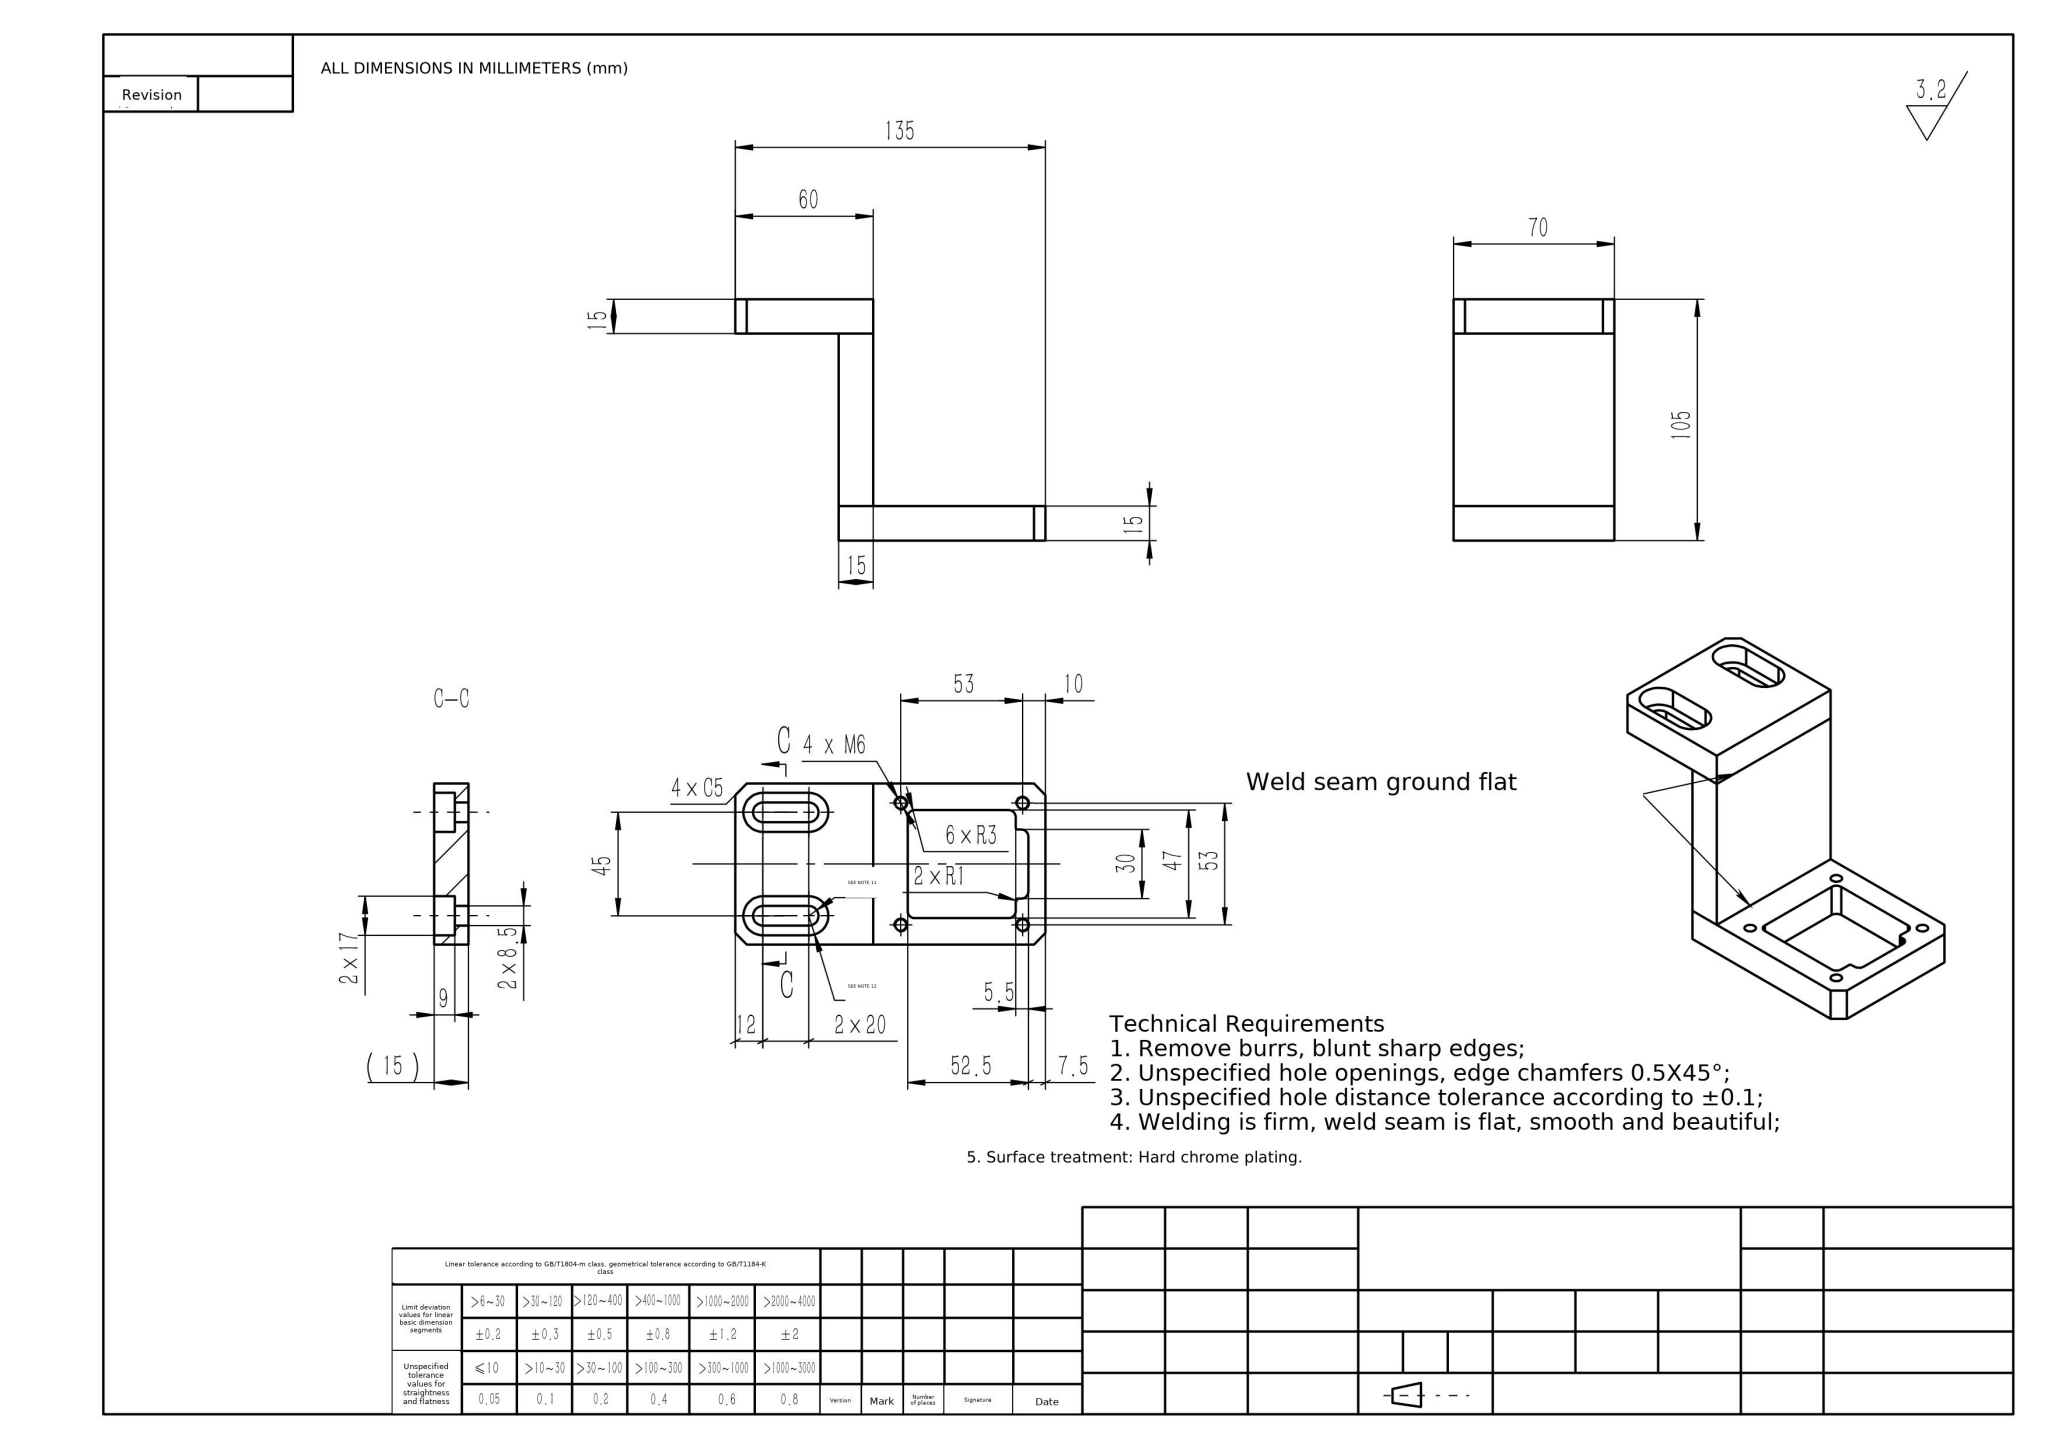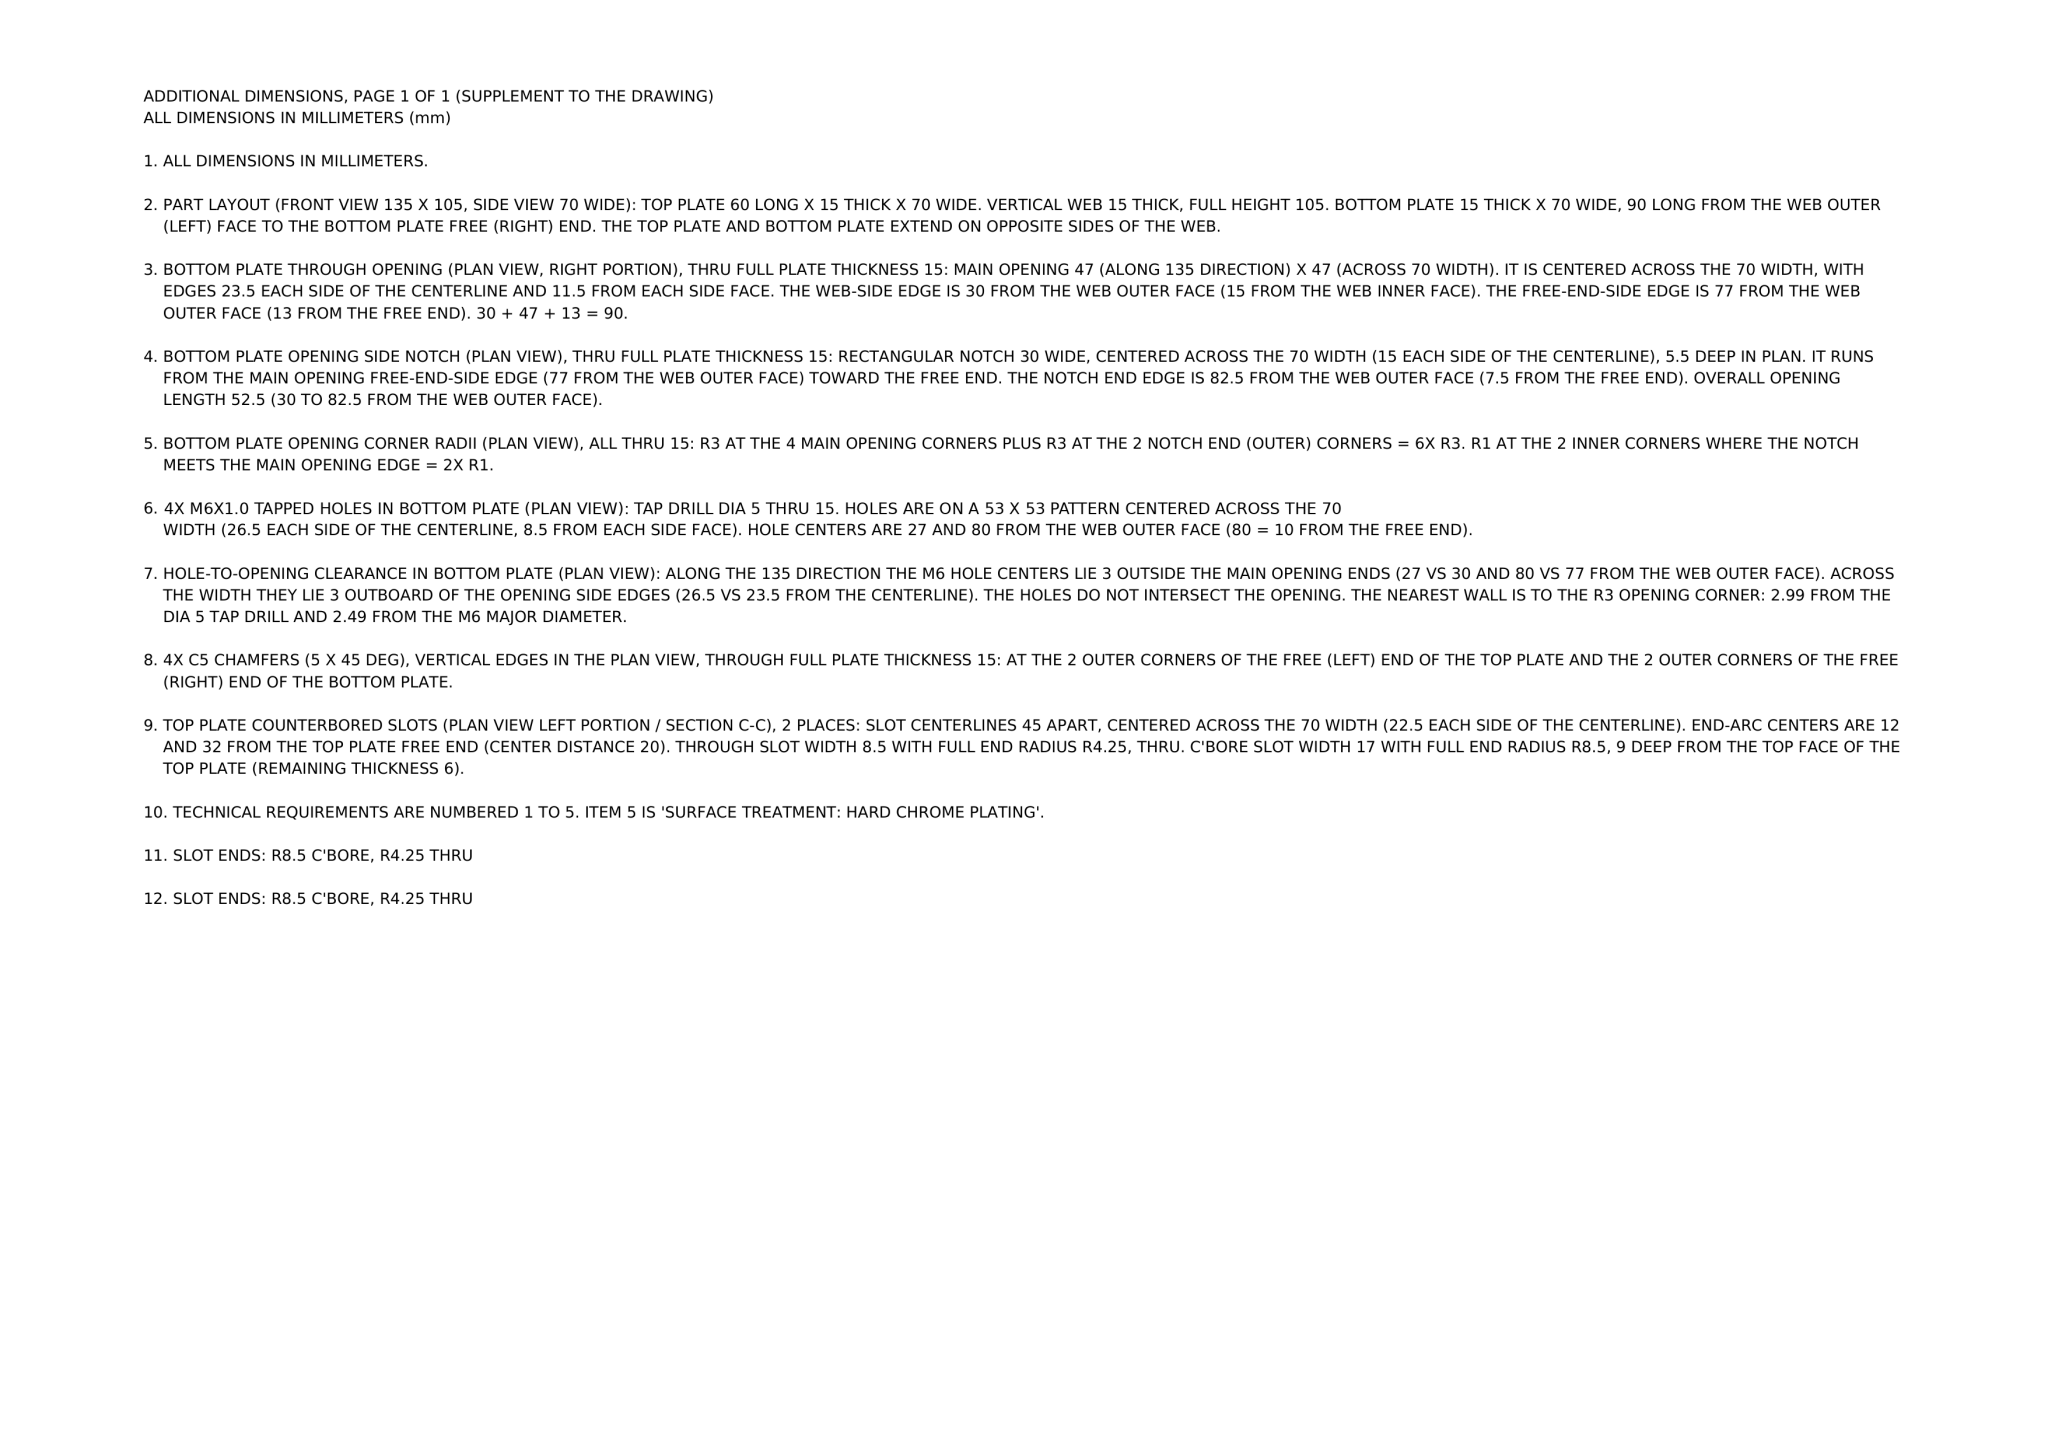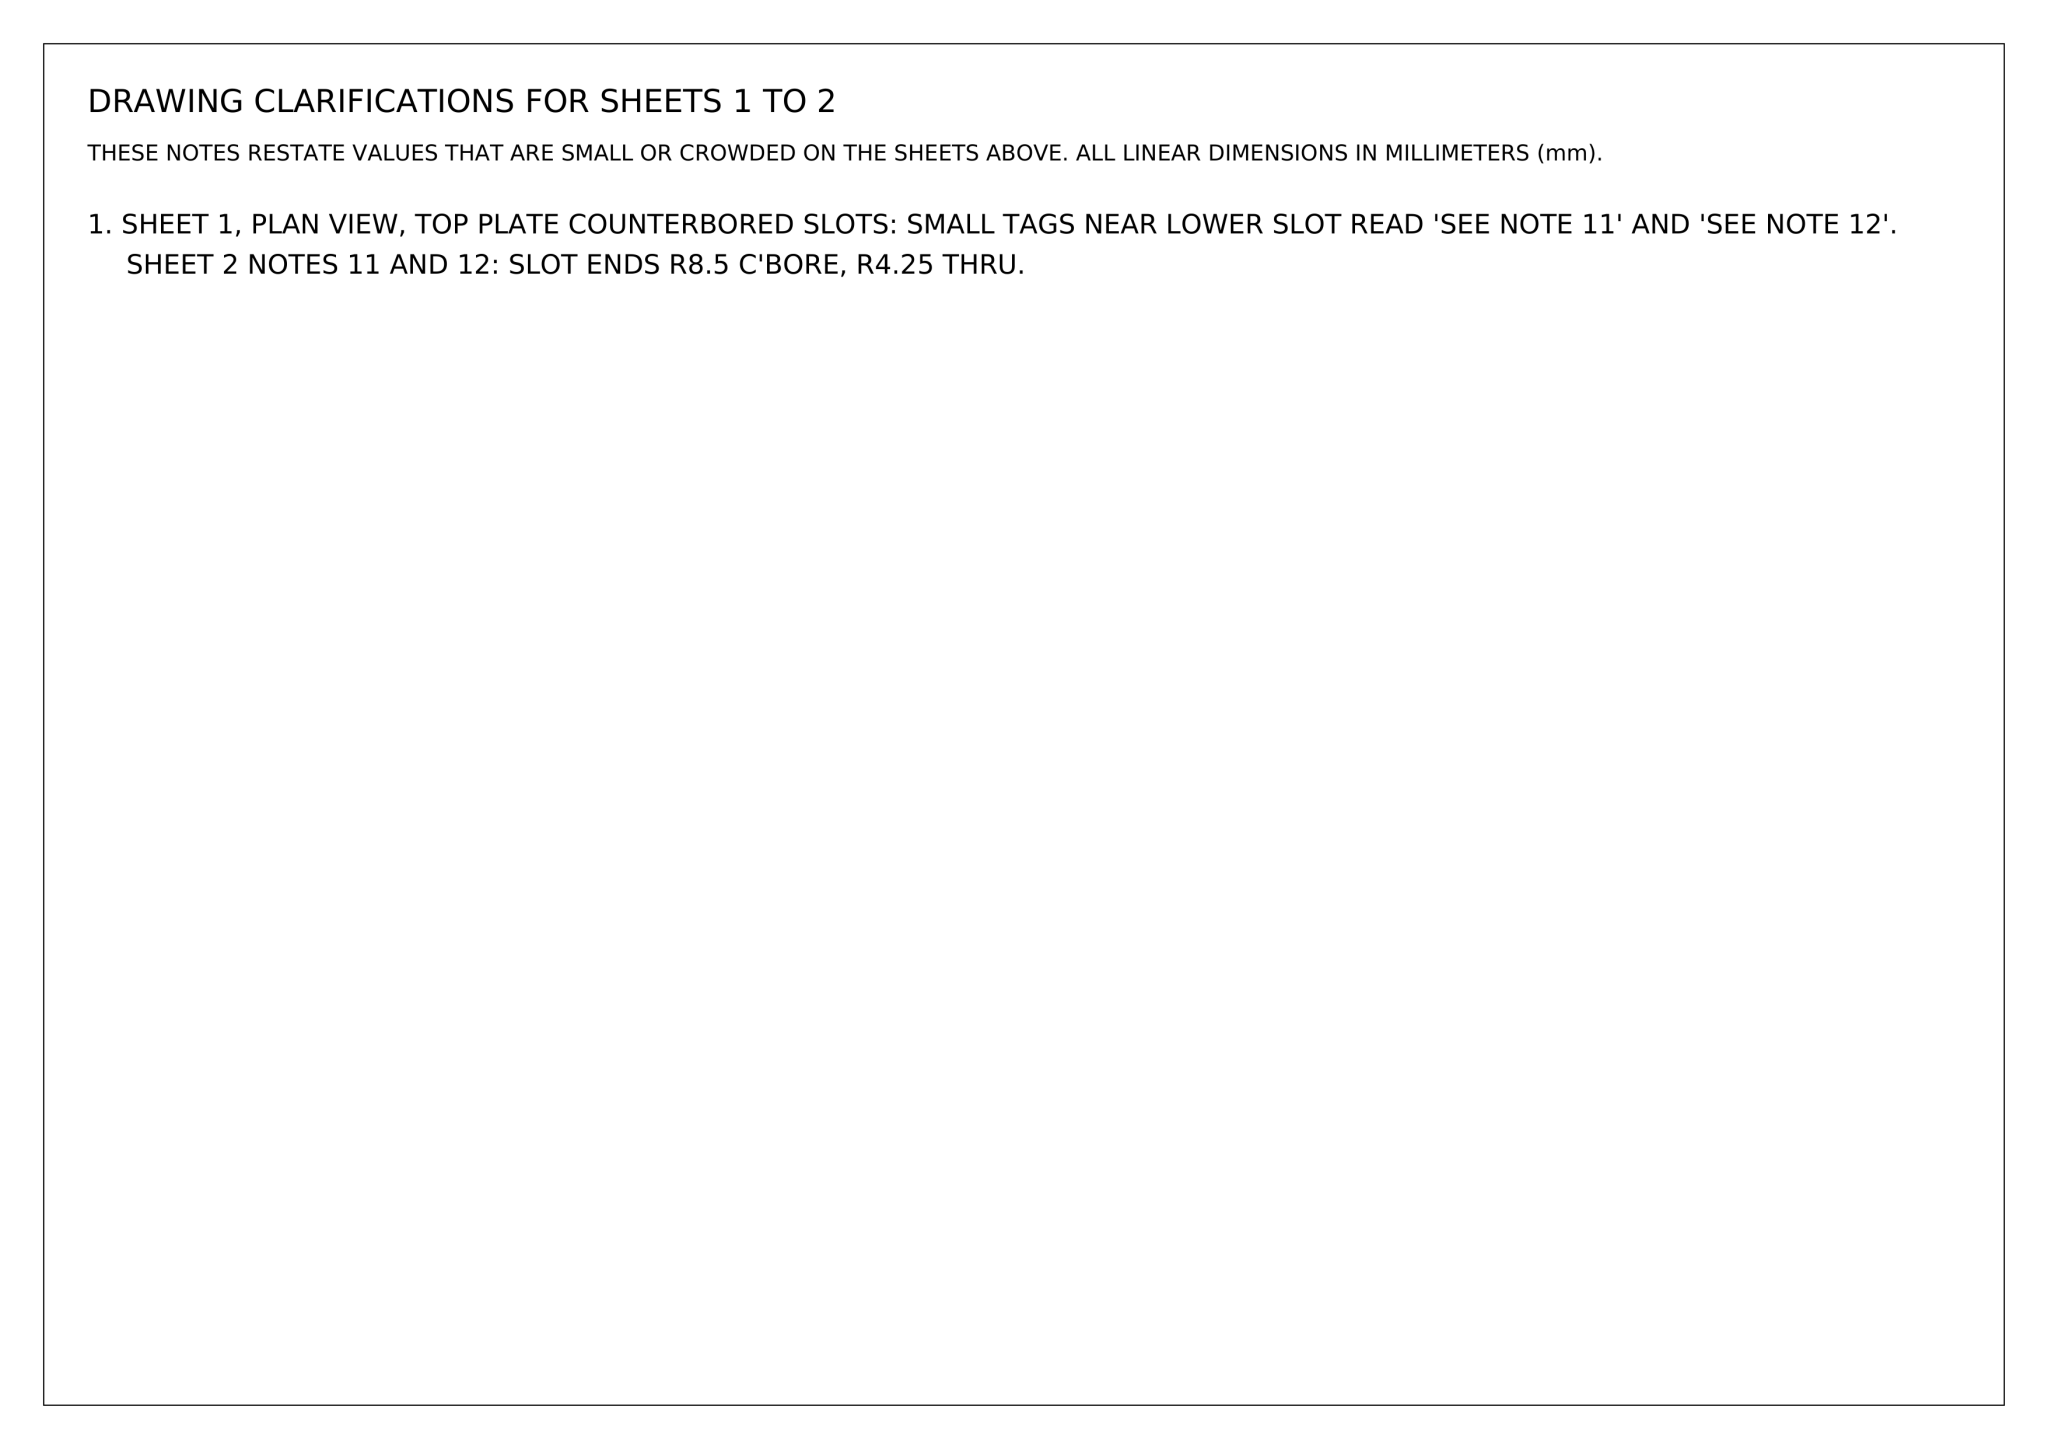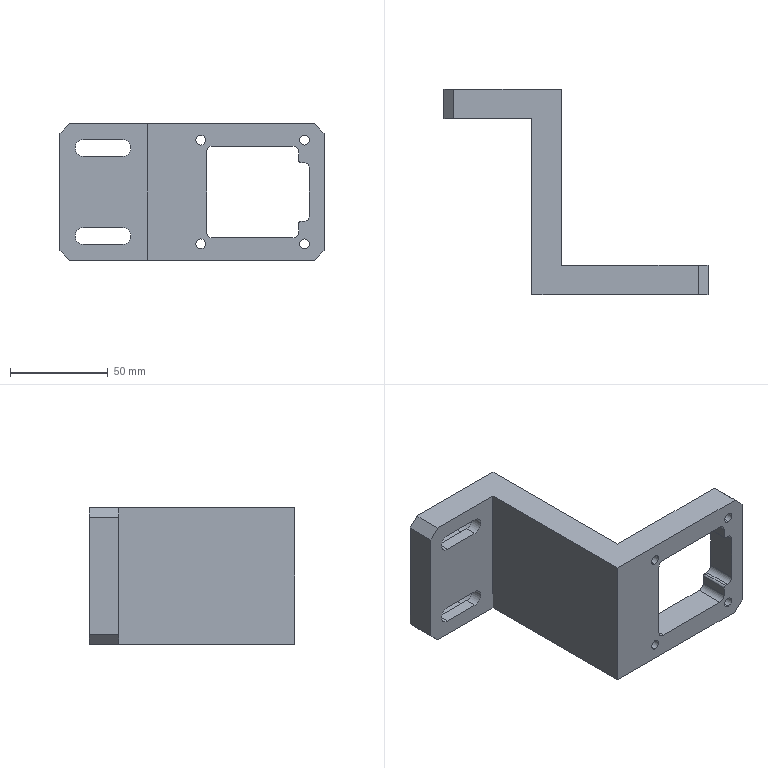Part | NX | mm | 1 solid | 60 faces | box 135 x 105 x 70 mm | volume 185953 mm3 | plane 32 | cylinder 28 | commonest cylinder face diameters 5 x8 17 x6 8.5 x6 6 x6 2 x2